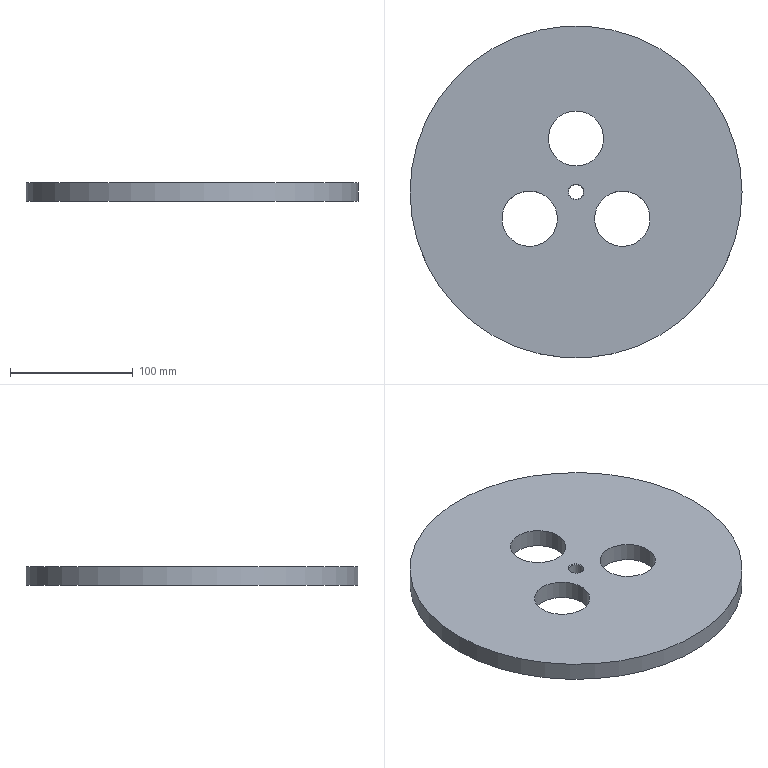Component | NX | EJECTOR_PLATE | 1 solid | 9 faces | box 270 x 270 x 15 mm | volume 785557 mm3 | cylinder 5 | plane 2 | cone 2 | commonest cylinder face diameters 45 x3 270 x1 12 x1
STEP:
#1=CARTESIAN_POINT('',(0.,0.,0.));
#2=DIRECTION('',(0.,0.,1.));
#3=DIRECTION('',(1.,0.,0.));
#4=AXIS2_PLACEMENT_3D('',#1,#2,#3);
#5=CARTESIAN_POINT('',(22.5,36.,213.));
#6=VERTEX_POINT('',#5);
#7=CARTESIAN_POINT('',(-0.,36.,213.));
#8=DIRECTION('',(0.,0.,1.));
#9=DIRECTION('',(1.,0.,0.));
#10=AXIS2_PLACEMENT_3D('',#7,#8,#9);
#11=CIRCLE('',#10,22.5);
#12=CARTESIAN_POINT('',(-0.,36.,213.));
#13=DIRECTION('',(0.,0.,-1.));
#14=DIRECTION('',(-1.,0.,0.));
#15=AXIS2_PLACEMENT_3D('',#12,#13,#14);
#16=CYLINDRICAL_SURFACE('',#15,22.5);
#17=CARTESIAN_POINT('',(9.425,0.));
#18=DIRECTION('',(-1.,0.));
#19=VECTOR('',#18,1.);
#20=LINE('',#17,#19);
#21=(GEOMETRIC_REPRESENTATION_CONTEXT(2)PARAMETRIC_REPRESENTATION_CONTEXT()REPRESENTATION_CONTEXT('',''));
#22=DEFINITIONAL_REPRESENTATION('',(#20),#21);
#23=PCURVE('',#16,#22);
#24=CARTESIAN_POINT('',(18.836,-18.375,213.));
#25=DIRECTION('',(0.,0.,1.));
#26=DIRECTION('',(1.,0.,0.));
#27=AXIS2_PLACEMENT_3D('',#24,#25,#26);
#28=PLANE('',#27);
#29=CARTESIAN_POINT('',(-18.836,54.375));
#30=DIRECTION('',(1.,0.));
#31=AXIS2_PLACEMENT_2D('',#29,#30);
#32=CIRCLE('',#31,22.5);
#33=(GEOMETRIC_REPRESENTATION_CONTEXT(2)PARAMETRIC_REPRESENTATION_CONTEXT()REPRESENTATION_CONTEXT('',''));
#34=DEFINITIONAL_REPRESENTATION('',(#32),#33);
#35=PCURVE('',#28,#34);
#36=SURFACE_CURVE('',#11,(#23,#35),.PCURVE_S1.);
#37=EDGE_CURVE('',#6,#6,#36,.T.);
#38=ORIENTED_EDGE('',*,*,#37,.F.);
#39=CARTESIAN_POINT('',(22.5,36.,198.));
#40=VERTEX_POINT('',#39);
#41=CARTESIAN_POINT('',(22.5,36.,213.));
#42=CARTESIAN_POINT('',(22.5,36.,198.));
#43=B_SPLINE_CURVE_WITH_KNOTS('',1,(#41,#42),.UNSPECIFIED.,.F.,.F.,(2,2),(0.,15.),.PIECEWISE_BEZIER_KNOTS.);
#44=CARTESIAN_POINT('',(9.425,0.));
#45=DIRECTION('',(0.,1.));
#46=VECTOR('',#45,1.);
#47=LINE('',#44,#46);
#48=(GEOMETRIC_REPRESENTATION_CONTEXT(2)PARAMETRIC_REPRESENTATION_CONTEXT()REPRESENTATION_CONTEXT('',''));
#49=DEFINITIONAL_REPRESENTATION('',(#47),#48);
#50=PCURVE('',#16,#49);
#51=CARTESIAN_POINT('',(3.142,0.));
#52=DIRECTION('',(0.,1.));
#53=VECTOR('',#52,1.);
#54=LINE('',#51,#53);
#55=(GEOMETRIC_REPRESENTATION_CONTEXT(2)PARAMETRIC_REPRESENTATION_CONTEXT()REPRESENTATION_CONTEXT('',''));
#56=DEFINITIONAL_REPRESENTATION('',(#54),#55);
#57=PCURVE('',#16,#56);
#58=SEAM_CURVE('',#43,(#50,#57),.PCURVE_S1.);
#59=EDGE_CURVE('',#6,#40,#58,.T.);
#60=ORIENTED_EDGE('',*,*,#59,.T.);
#61=CARTESIAN_POINT('',(-0.,36.,198.));
#62=DIRECTION('',(0.,0.,1.));
#63=DIRECTION('',(1.,0.,0.));
#64=AXIS2_PLACEMENT_3D('',#61,#62,#63);
#65=CIRCLE('',#64,22.5);
#66=CARTESIAN_POINT('',(9.425,15.));
#67=DIRECTION('',(-1.,0.));
#68=VECTOR('',#67,1.);
#69=LINE('',#66,#68);
#70=(GEOMETRIC_REPRESENTATION_CONTEXT(2)PARAMETRIC_REPRESENTATION_CONTEXT()REPRESENTATION_CONTEXT('',''));
#71=DEFINITIONAL_REPRESENTATION('',(#69),#70);
#72=PCURVE('',#16,#71);
#73=CARTESIAN_POINT('',(18.836,-18.375,198.));
#74=DIRECTION('',(0.,0.,1.));
#75=DIRECTION('',(1.,0.,0.));
#76=AXIS2_PLACEMENT_3D('',#73,#74,#75);
#77=PLANE('',#76);
#78=CARTESIAN_POINT('',(-18.836,54.375));
#79=DIRECTION('',(1.,0.));
#80=AXIS2_PLACEMENT_2D('',#78,#79);
#81=CIRCLE('',#80,22.5);
#82=(GEOMETRIC_REPRESENTATION_CONTEXT(2)PARAMETRIC_REPRESENTATION_CONTEXT()REPRESENTATION_CONTEXT('',''));
#83=DEFINITIONAL_REPRESENTATION('',(#81),#82);
#84=PCURVE('',#77,#83);
#85=SURFACE_CURVE('',#65,(#72,#84),.PCURVE_S1.);
#86=EDGE_CURVE('',#40,#40,#85,.T.);
#87=ORIENTED_EDGE('',*,*,#86,.T.);
#88=ORIENTED_EDGE('',*,*,#59,.F.);
#89=EDGE_LOOP('',(#38,#60,#87,#88));
#90=FACE_BOUND('',#89,.F.);
#91=ADVANCED_FACE('',(#90),#16,.F.);
#92=CARTESIAN_POINT('',(26.422,-48.736,213.));
#93=VERTEX_POINT('',#92);
#94=CARTESIAN_POINT('',(37.672,-29.25,213.));
#95=DIRECTION('',(0.,0.,1.));
#96=DIRECTION('',(-0.5,-0.866,0.));
#97=AXIS2_PLACEMENT_3D('',#94,#95,#96);
#98=CIRCLE('',#97,22.5);
#99=CARTESIAN_POINT('',(37.672,-29.25,213.));
#100=DIRECTION('',(0.,0.,-1.));
#101=DIRECTION('',(-1.,0.,0.));
#102=AXIS2_PLACEMENT_3D('',#99,#100,#101);
#103=CYLINDRICAL_SURFACE('',#102,22.5);
#104=CARTESIAN_POINT('',(11.519,0.));
#105=DIRECTION('',(-1.,0.));
#106=VECTOR('',#105,1.);
#107=LINE('',#104,#106);
#108=(GEOMETRIC_REPRESENTATION_CONTEXT(2)PARAMETRIC_REPRESENTATION_CONTEXT()REPRESENTATION_CONTEXT('',''));
#109=DEFINITIONAL_REPRESENTATION('',(#107),#108);
#110=PCURVE('',#103,#109);
#111=CARTESIAN_POINT('',(18.836,-10.875));
#112=DIRECTION('',(-0.5,-0.866));
#113=AXIS2_PLACEMENT_2D('',#111,#112);
#114=CIRCLE('',#113,22.5);
#115=(GEOMETRIC_REPRESENTATION_CONTEXT(2)PARAMETRIC_REPRESENTATION_CONTEXT()REPRESENTATION_CONTEXT('',''));
#116=DEFINITIONAL_REPRESENTATION('',(#114),#115);
#117=PCURVE('',#28,#116);
#118=SURFACE_CURVE('',#98,(#110,#117),.PCURVE_S1.);
#119=EDGE_CURVE('',#93,#93,#118,.T.);
#120=ORIENTED_EDGE('',*,*,#119,.F.);
#121=CARTESIAN_POINT('',(26.422,-48.736,198.));
#122=VERTEX_POINT('',#121);
#123=CARTESIAN_POINT('',(26.422,-48.736,213.));
#124=CARTESIAN_POINT('',(26.422,-48.736,198.));
#125=B_SPLINE_CURVE_WITH_KNOTS('',1,(#123,#124),.UNSPECIFIED.,.F.,.F.,(2,2),(0.,15.),.PIECEWISE_BEZIER_KNOTS.);
#126=CARTESIAN_POINT('',(11.519,0.));
#127=DIRECTION('',(0.,1.));
#128=VECTOR('',#127,1.);
#129=LINE('',#126,#128);
#130=(GEOMETRIC_REPRESENTATION_CONTEXT(2)PARAMETRIC_REPRESENTATION_CONTEXT()REPRESENTATION_CONTEXT('',''));
#131=DEFINITIONAL_REPRESENTATION('',(#129),#130);
#132=PCURVE('',#103,#131);
#133=CARTESIAN_POINT('',(5.236,0.));
#134=DIRECTION('',(0.,1.));
#135=VECTOR('',#134,1.);
#136=LINE('',#133,#135);
#137=(GEOMETRIC_REPRESENTATION_CONTEXT(2)PARAMETRIC_REPRESENTATION_CONTEXT()REPRESENTATION_CONTEXT('',''));
#138=DEFINITIONAL_REPRESENTATION('',(#136),#137);
#139=PCURVE('',#103,#138);
#140=SEAM_CURVE('',#125,(#132,#139),.PCURVE_S1.);
#141=EDGE_CURVE('',#93,#122,#140,.T.);
#142=ORIENTED_EDGE('',*,*,#141,.T.);
#143=CARTESIAN_POINT('',(37.672,-29.25,198.));
#144=DIRECTION('',(0.,0.,1.));
#145=DIRECTION('',(-0.5,-0.866,0.));
#146=AXIS2_PLACEMENT_3D('',#143,#144,#145);
#147=CIRCLE('',#146,22.5);
#148=CARTESIAN_POINT('',(11.519,15.));
#149=DIRECTION('',(-1.,0.));
#150=VECTOR('',#149,1.);
#151=LINE('',#148,#150);
#152=(GEOMETRIC_REPRESENTATION_CONTEXT(2)PARAMETRIC_REPRESENTATION_CONTEXT()REPRESENTATION_CONTEXT('',''));
#153=DEFINITIONAL_REPRESENTATION('',(#151),#152);
#154=PCURVE('',#103,#153);
#155=CARTESIAN_POINT('',(18.836,-10.875));
#156=DIRECTION('',(-0.5,-0.866));
#157=AXIS2_PLACEMENT_2D('',#155,#156);
#158=CIRCLE('',#157,22.5);
#159=(GEOMETRIC_REPRESENTATION_CONTEXT(2)PARAMETRIC_REPRESENTATION_CONTEXT()REPRESENTATION_CONTEXT('',''));
#160=DEFINITIONAL_REPRESENTATION('',(#158),#159);
#161=PCURVE('',#77,#160);
#162=SURFACE_CURVE('',#147,(#154,#161),.PCURVE_S1.);
#163=EDGE_CURVE('',#122,#122,#162,.T.);
#164=ORIENTED_EDGE('',*,*,#163,.T.);
#165=ORIENTED_EDGE('',*,*,#141,.F.);
#166=EDGE_LOOP('',(#120,#142,#164,#165));
#167=FACE_BOUND('',#166,.F.);
#168=ADVANCED_FACE('',(#167),#103,.F.);
#169=CARTESIAN_POINT('',(135.,-7.5,213.));
#170=VERTEX_POINT('',#169);
#171=CARTESIAN_POINT('',(-0.,-7.5,213.));
#172=DIRECTION('',(0.,0.,1.));
#173=DIRECTION('',(1.,0.,0.));
#174=AXIS2_PLACEMENT_3D('',#171,#172,#173);
#175=CIRCLE('',#174,135.);
#176=CARTESIAN_POINT('',(-0.,-7.5,213.));
#177=DIRECTION('',(0.,0.,-1.));
#178=DIRECTION('',(-1.,0.,0.));
#179=AXIS2_PLACEMENT_3D('',#176,#177,#178);
#180=CYLINDRICAL_SURFACE('',#179,135.);
#181=CARTESIAN_POINT('',(9.425,0.));
#182=DIRECTION('',(-1.,0.));
#183=VECTOR('',#182,1.);
#184=LINE('',#181,#183);
#185=(GEOMETRIC_REPRESENTATION_CONTEXT(2)PARAMETRIC_REPRESENTATION_CONTEXT()REPRESENTATION_CONTEXT('',''));
#186=DEFINITIONAL_REPRESENTATION('',(#184),#185);
#187=PCURVE('',#180,#186);
#188=CARTESIAN_POINT('',(-18.836,10.875));
#189=DIRECTION('',(1.,0.));
#190=AXIS2_PLACEMENT_2D('',#188,#189);
#191=CIRCLE('',#190,135.);
#192=(GEOMETRIC_REPRESENTATION_CONTEXT(2)PARAMETRIC_REPRESENTATION_CONTEXT()REPRESENTATION_CONTEXT('',''));
#193=DEFINITIONAL_REPRESENTATION('',(#191),#192);
#194=PCURVE('',#28,#193);
#195=SURFACE_CURVE('',#175,(#187,#194),.PCURVE_S1.);
#196=EDGE_CURVE('',#170,#170,#195,.T.);
#197=ORIENTED_EDGE('',*,*,#196,.F.);
#198=CARTESIAN_POINT('',(135.,-7.5,198.));
#199=VERTEX_POINT('',#198);
#200=CARTESIAN_POINT('',(135.,-7.5,213.));
#201=CARTESIAN_POINT('',(135.,-7.5,198.));
#202=B_SPLINE_CURVE_WITH_KNOTS('',1,(#200,#201),.UNSPECIFIED.,.F.,.F.,(2,2),(0.,15.),.PIECEWISE_BEZIER_KNOTS.);
#203=CARTESIAN_POINT('',(9.425,0.));
#204=DIRECTION('',(0.,1.));
#205=VECTOR('',#204,1.);
#206=LINE('',#203,#205);
#207=(GEOMETRIC_REPRESENTATION_CONTEXT(2)PARAMETRIC_REPRESENTATION_CONTEXT()REPRESENTATION_CONTEXT('',''));
#208=DEFINITIONAL_REPRESENTATION('',(#206),#207);
#209=PCURVE('',#180,#208);
#210=CARTESIAN_POINT('',(3.142,0.));
#211=DIRECTION('',(0.,1.));
#212=VECTOR('',#211,1.);
#213=LINE('',#210,#212);
#214=(GEOMETRIC_REPRESENTATION_CONTEXT(2)PARAMETRIC_REPRESENTATION_CONTEXT()REPRESENTATION_CONTEXT('',''));
#215=DEFINITIONAL_REPRESENTATION('',(#213),#214);
#216=PCURVE('',#180,#215);
#217=SEAM_CURVE('',#202,(#209,#216),.PCURVE_S1.);
#218=EDGE_CURVE('',#170,#199,#217,.T.);
#219=ORIENTED_EDGE('',*,*,#218,.T.);
#220=CARTESIAN_POINT('',(-0.,-7.5,198.));
#221=DIRECTION('',(0.,0.,1.));
#222=DIRECTION('',(1.,0.,0.));
#223=AXIS2_PLACEMENT_3D('',#220,#221,#222);
#224=CIRCLE('',#223,135.);
#225=CARTESIAN_POINT('',(9.425,15.));
#226=DIRECTION('',(-1.,0.));
#227=VECTOR('',#226,1.);
#228=LINE('',#225,#227);
#229=(GEOMETRIC_REPRESENTATION_CONTEXT(2)PARAMETRIC_REPRESENTATION_CONTEXT()REPRESENTATION_CONTEXT('',''));
#230=DEFINITIONAL_REPRESENTATION('',(#228),#229);
#231=PCURVE('',#180,#230);
#232=CARTESIAN_POINT('',(-18.836,10.875));
#233=DIRECTION('',(1.,0.));
#234=AXIS2_PLACEMENT_2D('',#232,#233);
#235=CIRCLE('',#234,135.);
#236=(GEOMETRIC_REPRESENTATION_CONTEXT(2)PARAMETRIC_REPRESENTATION_CONTEXT()REPRESENTATION_CONTEXT('',''));
#237=DEFINITIONAL_REPRESENTATION('',(#235),#236);
#238=PCURVE('',#77,#237);
#239=SURFACE_CURVE('',#224,(#231,#238),.PCURVE_S1.);
#240=EDGE_CURVE('',#199,#199,#239,.T.);
#241=ORIENTED_EDGE('',*,*,#240,.T.);
#242=ORIENTED_EDGE('',*,*,#218,.F.);
#243=EDGE_LOOP('',(#197,#219,#241,#242));
#244=FACE_BOUND('',#243,.T.);
#245=ADVANCED_FACE('',(#244),#180,.T.);
#246=CARTESIAN_POINT('',(-48.922,-9.764,213.));
#247=VERTEX_POINT('',#246);
#248=CARTESIAN_POINT('',(-37.672,-29.25,213.));
#249=DIRECTION('',(0.,0.,1.));
#250=DIRECTION('',(-0.5,0.866,0.));
#251=AXIS2_PLACEMENT_3D('',#248,#249,#250);
#252=CIRCLE('',#251,22.5);
#253=CARTESIAN_POINT('',(-37.672,-29.25,213.));
#254=DIRECTION('',(0.,0.,-1.));
#255=DIRECTION('',(-1.,0.,0.));
#256=AXIS2_PLACEMENT_3D('',#253,#254,#255);
#257=CYLINDRICAL_SURFACE('',#256,22.5);
#258=CARTESIAN_POINT('',(7.33,0.));
#259=DIRECTION('',(-1.,0.));
#260=VECTOR('',#259,1.);
#261=LINE('',#258,#260);
#262=(GEOMETRIC_REPRESENTATION_CONTEXT(2)PARAMETRIC_REPRESENTATION_CONTEXT()REPRESENTATION_CONTEXT('',''));
#263=DEFINITIONAL_REPRESENTATION('',(#261),#262);
#264=PCURVE('',#257,#263);
#265=CARTESIAN_POINT('',(-56.508,-10.875));
#266=DIRECTION('',(-0.5,0.866));
#267=AXIS2_PLACEMENT_2D('',#265,#266);
#268=CIRCLE('',#267,22.5);
#269=(GEOMETRIC_REPRESENTATION_CONTEXT(2)PARAMETRIC_REPRESENTATION_CONTEXT()REPRESENTATION_CONTEXT('',''));
#270=DEFINITIONAL_REPRESENTATION('',(#268),#269);
#271=PCURVE('',#28,#270);
#272=SURFACE_CURVE('',#252,(#264,#271),.PCURVE_S1.);
#273=EDGE_CURVE('',#247,#247,#272,.T.);
#274=ORIENTED_EDGE('',*,*,#273,.F.);
#275=CARTESIAN_POINT('',(-48.922,-9.764,198.));
#276=VERTEX_POINT('',#275);
#277=CARTESIAN_POINT('',(-48.922,-9.764,213.));
#278=CARTESIAN_POINT('',(-48.922,-9.764,198.));
#279=B_SPLINE_CURVE_WITH_KNOTS('',1,(#277,#278),.UNSPECIFIED.,.F.,.F.,(2,2),(0.,15.),.PIECEWISE_BEZIER_KNOTS.);
#280=CARTESIAN_POINT('',(7.33,0.));
#281=DIRECTION('',(0.,1.));
#282=VECTOR('',#281,1.);
#283=LINE('',#280,#282);
#284=(GEOMETRIC_REPRESENTATION_CONTEXT(2)PARAMETRIC_REPRESENTATION_CONTEXT()REPRESENTATION_CONTEXT('',''));
#285=DEFINITIONAL_REPRESENTATION('',(#283),#284);
#286=PCURVE('',#257,#285);
#287=CARTESIAN_POINT('',(1.047,0.));
#288=DIRECTION('',(0.,1.));
#289=VECTOR('',#288,1.);
#290=LINE('',#287,#289);
#291=(GEOMETRIC_REPRESENTATION_CONTEXT(2)PARAMETRIC_REPRESENTATION_CONTEXT()REPRESENTATION_CONTEXT('',''));
#292=DEFINITIONAL_REPRESENTATION('',(#290),#291);
#293=PCURVE('',#257,#292);
#294=SEAM_CURVE('',#279,(#286,#293),.PCURVE_S1.);
#295=EDGE_CURVE('',#247,#276,#294,.T.);
#296=ORIENTED_EDGE('',*,*,#295,.T.);
#297=CARTESIAN_POINT('',(-37.672,-29.25,198.));
#298=DIRECTION('',(0.,0.,1.));
#299=DIRECTION('',(-0.5,0.866,0.));
#300=AXIS2_PLACEMENT_3D('',#297,#298,#299);
#301=CIRCLE('',#300,22.5);
#302=CARTESIAN_POINT('',(7.33,15.));
#303=DIRECTION('',(-1.,0.));
#304=VECTOR('',#303,1.);
#305=LINE('',#302,#304);
#306=(GEOMETRIC_REPRESENTATION_CONTEXT(2)PARAMETRIC_REPRESENTATION_CONTEXT()REPRESENTATION_CONTEXT('',''));
#307=DEFINITIONAL_REPRESENTATION('',(#305),#306);
#308=PCURVE('',#257,#307);
#309=CARTESIAN_POINT('',(-56.508,-10.875));
#310=DIRECTION('',(-0.5,0.866));
#311=AXIS2_PLACEMENT_2D('',#309,#310);
#312=CIRCLE('',#311,22.5);
#313=(GEOMETRIC_REPRESENTATION_CONTEXT(2)PARAMETRIC_REPRESENTATION_CONTEXT()REPRESENTATION_CONTEXT('',''));
#314=DEFINITIONAL_REPRESENTATION('',(#312),#313);
#315=PCURVE('',#77,#314);
#316=SURFACE_CURVE('',#301,(#308,#315),.PCURVE_S1.);
#317=EDGE_CURVE('',#276,#276,#316,.T.);
#318=ORIENTED_EDGE('',*,*,#317,.T.);
#319=ORIENTED_EDGE('',*,*,#295,.F.);
#320=EDGE_LOOP('',(#274,#296,#318,#319));
#321=FACE_BOUND('',#320,.F.);
#322=ADVANCED_FACE('',(#321),#257,.F.);
#323=CARTESIAN_POINT('',(6.5,-7.5,213.));
#324=VERTEX_POINT('',#323);
#325=CARTESIAN_POINT('',(-0.,-7.5,213.));
#326=DIRECTION('',(0.,0.,-1.));
#327=DIRECTION('',(1.,0.,0.));
#328=AXIS2_PLACEMENT_3D('',#325,#326,#327);
#329=CIRCLE('',#328,6.5);
#330=CARTESIAN_POINT('',(-12.336,10.875));
#331=CARTESIAN_POINT('',(-12.336,-0.3833));
#332=CARTESIAN_POINT('',(-22.086,5.246));
#333=CARTESIAN_POINT('',(-31.836,10.875));
#334=CARTESIAN_POINT('',(-22.086,16.504));
#335=CARTESIAN_POINT('',(-12.336,22.133));
#336=CARTESIAN_POINT('',(-12.336,10.875));
#337=(BOUNDED_CURVE()B_SPLINE_CURVE(2,(#330,#331,#332,#333,#334,#335,#336),.UNSPECIFIED.,.T.,.F.)B_SPLINE_CURVE_WITH_KNOTS((1,2,2,2,2,1),(-2.094,0.,2.094,4.189,6.283,8.378),.UNSPECIFIED.)CURVE()GEOMETRIC_REPRESENTATION_ITEM()RATIONAL_B_SPLINE_CURVE((1.,0.5,1.,0.5,1.,0.5,1.))REPRESENTATION_ITEM(''));
#338=(GEOMETRIC_REPRESENTATION_CONTEXT(2)PARAMETRIC_REPRESENTATION_CONTEXT()REPRESENTATION_CONTEXT('',''));
#339=DEFINITIONAL_REPRESENTATION('',(#337),#338);
#340=PCURVE('',#28,#339);
#341=CARTESIAN_POINT('',(-0.,-7.5,213.));
#342=DIRECTION('',(0.,0.,1.));
#343=DIRECTION('',(1.,0.,0.));
#344=AXIS2_PLACEMENT_3D('',#341,#342,#343);
#345=CONICAL_SURFACE('',#344,6.5,0.7854);
#346=CARTESIAN_POINT('',(6.283,0.));
#347=DIRECTION('',(-1.,0.));
#348=VECTOR('',#347,1.);
#349=LINE('',#346,#348);
#350=(GEOMETRIC_REPRESENTATION_CONTEXT(2)PARAMETRIC_REPRESENTATION_CONTEXT()REPRESENTATION_CONTEXT('',''));
#351=DEFINITIONAL_REPRESENTATION('',(#349),#350);
#352=PCURVE('',#345,#351);
#353=SURFACE_CURVE('',#329,(#340,#352),.PCURVE_S1.);
#354=EDGE_CURVE('',#324,#324,#353,.T.);
#355=ORIENTED_EDGE('',*,*,#354,.T.);
#356=EDGE_LOOP('',(#355));
#357=FACE_BOUND('',#356,.T.);
#358=ORIENTED_EDGE('',*,*,#196,.T.);
#359=EDGE_LOOP('',(#358));
#360=FACE_BOUND('',#359,.T.);
#361=ORIENTED_EDGE('',*,*,#119,.F.);
#362=EDGE_LOOP('',(#361));
#363=FACE_BOUND('',#362,.T.);
#364=ORIENTED_EDGE('',*,*,#37,.F.);
#365=EDGE_LOOP('',(#364));
#366=FACE_BOUND('',#365,.T.);
#367=ORIENTED_EDGE('',*,*,#273,.F.);
#368=EDGE_LOOP('',(#367));
#369=FACE_BOUND('',#368,.T.);
#370=ADVANCED_FACE('',(#357,#360,#363,#366,#369),#28,.T.);
#371=CARTESIAN_POINT('',(6.5,-7.5,198.));
#372=VERTEX_POINT('',#371);
#373=CARTESIAN_POINT('',(-0.,-7.5,198.));
#374=DIRECTION('',(0.,0.,1.));
#375=DIRECTION('',(1.,0.,0.));
#376=AXIS2_PLACEMENT_3D('',#373,#374,#375);
#377=CIRCLE('',#376,6.5);
#378=CARTESIAN_POINT('',(-18.836,10.875));
#379=DIRECTION('',(1.,0.));
#380=AXIS2_PLACEMENT_2D('',#378,#379);
#381=CIRCLE('',#380,6.5);
#382=(GEOMETRIC_REPRESENTATION_CONTEXT(2)PARAMETRIC_REPRESENTATION_CONTEXT()REPRESENTATION_CONTEXT('',''));
#383=DEFINITIONAL_REPRESENTATION('',(#381),#382);
#384=PCURVE('',#77,#383);
#385=CARTESIAN_POINT('',(-0.,-7.5,198.));
#386=DIRECTION('',(0.,0.,-1.));
#387=DIRECTION('',(-1.,0.,0.));
#388=AXIS2_PLACEMENT_3D('',#385,#386,#387);
#389=CONICAL_SURFACE('',#388,6.5,0.7854);
#390=CARTESIAN_POINT('',(9.425,0.));
#391=DIRECTION('',(-1.,0.));
#392=VECTOR('',#391,1.);
#393=LINE('',#390,#392);
#394=(GEOMETRIC_REPRESENTATION_CONTEXT(2)PARAMETRIC_REPRESENTATION_CONTEXT()REPRESENTATION_CONTEXT('',''));
#395=DEFINITIONAL_REPRESENTATION('',(#393),#394);
#396=PCURVE('',#389,#395);
#397=SURFACE_CURVE('',#377,(#384,#396),.PCURVE_S1.);
#398=EDGE_CURVE('',#372,#372,#397,.T.);
#399=ORIENTED_EDGE('',*,*,#398,.T.);
#400=EDGE_LOOP('',(#399));
#401=FACE_BOUND('',#400,.T.);
#402=ORIENTED_EDGE('',*,*,#240,.F.);
#403=EDGE_LOOP('',(#402));
#404=FACE_BOUND('',#403,.T.);
#405=ORIENTED_EDGE('',*,*,#163,.T.);
#406=EDGE_LOOP('',(#405));
#407=FACE_BOUND('',#406,.T.);
#408=ORIENTED_EDGE('',*,*,#86,.T.);
#409=EDGE_LOOP('',(#408));
#410=FACE_BOUND('',#409,.T.);
#411=ORIENTED_EDGE('',*,*,#317,.T.);
#412=EDGE_LOOP('',(#411));
#413=FACE_BOUND('',#412,.T.);
#414=ADVANCED_FACE('',(#401,#404,#407,#410,#413),#77,.F.);
#415=CARTESIAN_POINT('',(6.,-7.5,198.5));
#416=VERTEX_POINT('',#415);
#417=CARTESIAN_POINT('',(-0.,-7.5,198.5));
#418=DIRECTION('',(0.,0.,-1.));
#419=DIRECTION('',(1.,0.,0.));
#420=AXIS2_PLACEMENT_3D('',#417,#418,#419);
#421=CIRCLE('',#420,6.);
#422=CARTESIAN_POINT('',(-0.,-7.5,213.));
#423=DIRECTION('',(0.,0.,-1.));
#424=DIRECTION('',(-1.,0.,0.));
#425=AXIS2_PLACEMENT_3D('',#422,#423,#424);
#426=CYLINDRICAL_SURFACE('',#425,6.);
#427=CARTESIAN_POINT('',(3.142,14.5));
#428=DIRECTION('',(1.,0.));
#429=VECTOR('',#428,1.);
#430=LINE('',#427,#429);
#431=(GEOMETRIC_REPRESENTATION_CONTEXT(2)PARAMETRIC_REPRESENTATION_CONTEXT()REPRESENTATION_CONTEXT('',''));
#432=DEFINITIONAL_REPRESENTATION('',(#430),#431);
#433=PCURVE('',#426,#432);
#434=CARTESIAN_POINT('',(3.142,-0.5));
#435=DIRECTION('',(1.,0.));
#436=VECTOR('',#435,1.);
#437=LINE('',#434,#436);
#438=(GEOMETRIC_REPRESENTATION_CONTEXT(2)PARAMETRIC_REPRESENTATION_CONTEXT()REPRESENTATION_CONTEXT('',''));
#439=DEFINITIONAL_REPRESENTATION('',(#437),#438);
#440=PCURVE('',#389,#439);
#441=SURFACE_CURVE('',#421,(#433,#440),.PCURVE_S1.);
#442=EDGE_CURVE('',#416,#416,#441,.T.);
#443=ORIENTED_EDGE('',*,*,#442,.F.);
#444=CARTESIAN_POINT('',(6.,-7.5,212.5));
#445=VERTEX_POINT('',#444);
#446=CARTESIAN_POINT('',(6.,-7.5,212.5));
#447=CARTESIAN_POINT('',(6.,-7.5,198.5));
#448=B_SPLINE_CURVE_WITH_KNOTS('',1,(#446,#447),.UNSPECIFIED.,.F.,.F.,(2,2),(0.5,14.5),.PIECEWISE_BEZIER_KNOTS.);
#449=CARTESIAN_POINT('',(3.142,0.));
#450=DIRECTION('',(0.,1.));
#451=VECTOR('',#450,1.);
#452=LINE('',#449,#451);
#453=(GEOMETRIC_REPRESENTATION_CONTEXT(2)PARAMETRIC_REPRESENTATION_CONTEXT()REPRESENTATION_CONTEXT('',''));
#454=DEFINITIONAL_REPRESENTATION('',(#452),#453);
#455=PCURVE('',#426,#454);
#456=CARTESIAN_POINT('',(9.425,0.));
#457=DIRECTION('',(0.,1.));
#458=VECTOR('',#457,1.);
#459=LINE('',#456,#458);
#460=(GEOMETRIC_REPRESENTATION_CONTEXT(2)PARAMETRIC_REPRESENTATION_CONTEXT()REPRESENTATION_CONTEXT('',''));
#461=DEFINITIONAL_REPRESENTATION('',(#459),#460);
#462=PCURVE('',#426,#461);
#463=SEAM_CURVE('',#448,(#455,#462),.PCURVE_S1.);
#464=EDGE_CURVE('',#445,#416,#463,.T.);
#465=ORIENTED_EDGE('',*,*,#464,.F.);
#466=CARTESIAN_POINT('',(-0.,-7.5,212.5));
#467=DIRECTION('',(0.,0.,1.));
#468=DIRECTION('',(1.,0.,0.));
#469=AXIS2_PLACEMENT_3D('',#466,#467,#468);
#470=CIRCLE('',#469,6.);
#471=CARTESIAN_POINT('',(9.425,0.5));
#472=DIRECTION('',(-1.,0.));
#473=VECTOR('',#472,1.);
#474=LINE('',#471,#473);
#475=(GEOMETRIC_REPRESENTATION_CONTEXT(2)PARAMETRIC_REPRESENTATION_CONTEXT()REPRESENTATION_CONTEXT('',''));
#476=DEFINITIONAL_REPRESENTATION('',(#474),#475);
#477=PCURVE('',#426,#476);
#478=CARTESIAN_POINT('',(0.,-0.5));
#479=DIRECTION('',(1.,0.));
#480=VECTOR('',#479,1.);
#481=LINE('',#478,#480);
#482=(GEOMETRIC_REPRESENTATION_CONTEXT(2)PARAMETRIC_REPRESENTATION_CONTEXT()REPRESENTATION_CONTEXT('',''));
#483=DEFINITIONAL_REPRESENTATION('',(#481),#482);
#484=PCURVE('',#345,#483);
#485=SURFACE_CURVE('',#470,(#477,#484),.PCURVE_S1.);
#486=EDGE_CURVE('',#445,#445,#485,.T.);
#487=ORIENTED_EDGE('',*,*,#486,.F.);
#488=ORIENTED_EDGE('',*,*,#464,.T.);
#489=EDGE_LOOP('',(#443,#465,#487,#488));
#490=FACE_BOUND('',#489,.F.);
#491=ADVANCED_FACE('',(#490),#426,.F.);
#492=ORIENTED_EDGE('',*,*,#486,.T.);
#493=CARTESIAN_POINT('',(6.,-7.5,212.5));
#494=CARTESIAN_POINT('',(6.5,-7.5,213.));
#495=B_SPLINE_CURVE_WITH_KNOTS('',1,(#493,#494),.UNSPECIFIED.,.F.,.F.,(2,2),(-0.7071,0.),.PIECEWISE_BEZIER_KNOTS.);
#496=CARTESIAN_POINT('',(6.283,0.));
#497=DIRECTION('',(0.,1.));
#498=VECTOR('',#497,1.);
#499=LINE('',#496,#498);
#500=(GEOMETRIC_REPRESENTATION_CONTEXT(2)PARAMETRIC_REPRESENTATION_CONTEXT()REPRESENTATION_CONTEXT('',''));
#501=DEFINITIONAL_REPRESENTATION('',(#499),#500);
#502=PCURVE('',#345,#501);
#503=CARTESIAN_POINT('',(0.,0.));
#504=DIRECTION('',(0.,1.));
#505=VECTOR('',#504,1.);
#506=LINE('',#503,#505);
#507=(GEOMETRIC_REPRESENTATION_CONTEXT(2)PARAMETRIC_REPRESENTATION_CONTEXT()REPRESENTATION_CONTEXT('',''));
#508=DEFINITIONAL_REPRESENTATION('',(#506),#507);
#509=PCURVE('',#345,#508);
#510=SEAM_CURVE('',#495,(#502,#509),.PCURVE_S1.);
#511=EDGE_CURVE('',#445,#324,#510,.T.);
#512=ORIENTED_EDGE('',*,*,#511,.T.);
#513=ORIENTED_EDGE('',*,*,#354,.T.);
#514=ORIENTED_EDGE('',*,*,#511,.F.);
#515=EDGE_LOOP('',(#492,#512,#513,#514));
#516=FACE_BOUND('',#515,.F.);
#517=ADVANCED_FACE('',(#516),#345,.F.);
#518=ORIENTED_EDGE('',*,*,#442,.T.);
#519=CARTESIAN_POINT('',(6.,-7.5,198.5));
#520=CARTESIAN_POINT('',(6.5,-7.5,198.));
#521=B_SPLINE_CURVE_WITH_KNOTS('',1,(#519,#520),.UNSPECIFIED.,.F.,.F.,(2,2),(-0.7071,0.),.PIECEWISE_BEZIER_KNOTS.);
#522=CARTESIAN_POINT('',(9.425,0.));
#523=DIRECTION('',(0.,1.));
#524=VECTOR('',#523,1.);
#525=LINE('',#522,#524);
#526=(GEOMETRIC_REPRESENTATION_CONTEXT(2)PARAMETRIC_REPRESENTATION_CONTEXT()REPRESENTATION_CONTEXT('',''));
#527=DEFINITIONAL_REPRESENTATION('',(#525),#526);
#528=PCURVE('',#389,#527);
#529=CARTESIAN_POINT('',(3.142,0.));
#530=DIRECTION('',(0.,1.));
#531=VECTOR('',#530,1.);
#532=LINE('',#529,#531);
#533=(GEOMETRIC_REPRESENTATION_CONTEXT(2)PARAMETRIC_REPRESENTATION_CONTEXT()REPRESENTATION_CONTEXT('',''));
#534=DEFINITIONAL_REPRESENTATION('',(#532),#533);
#535=PCURVE('',#389,#534);
#536=SEAM_CURVE('',#521,(#528,#535),.PCURVE_S1.);
#537=EDGE_CURVE('',#416,#372,#536,.T.);
#538=ORIENTED_EDGE('',*,*,#537,.T.);
#539=ORIENTED_EDGE('',*,*,#398,.T.);
#540=ORIENTED_EDGE('',*,*,#537,.F.);
#541=EDGE_LOOP('',(#518,#538,#539,#540));
#542=FACE_BOUND('',#541,.F.);
#543=ADVANCED_FACE('',(#542),#389,.F.);
#544=CLOSED_SHELL('',(#91,#168,#245,#322,#370,#414,#491,#517,#543));
#545=MANIFOLD_SOLID_BREP('',#544);
#546=(LENGTH_UNIT()NAMED_UNIT(*)SI_UNIT(.MILLI.,.METRE.));
#547=UNCERTAINTY_MEASURE_WITH_UNIT(LENGTH_MEASURE(0.00001),#546,'','');
#548=(NAMED_UNIT(*)PLANE_ANGLE_UNIT()SI_UNIT($,.RADIAN.));
#549=(NAMED_UNIT(*)SI_UNIT($,.STERADIAN.)SOLID_ANGLE_UNIT());
#550=(GEOMETRIC_REPRESENTATION_CONTEXT(3)GLOBAL_UNCERTAINTY_ASSIGNED_CONTEXT((#547))GLOBAL_UNIT_ASSIGNED_CONTEXT((#546,#548,#549))REPRESENTATION_CONTEXT('',''));
#551=ADVANCED_BREP_SHAPE_REPRESENTATION('',(#4,#545),#550);